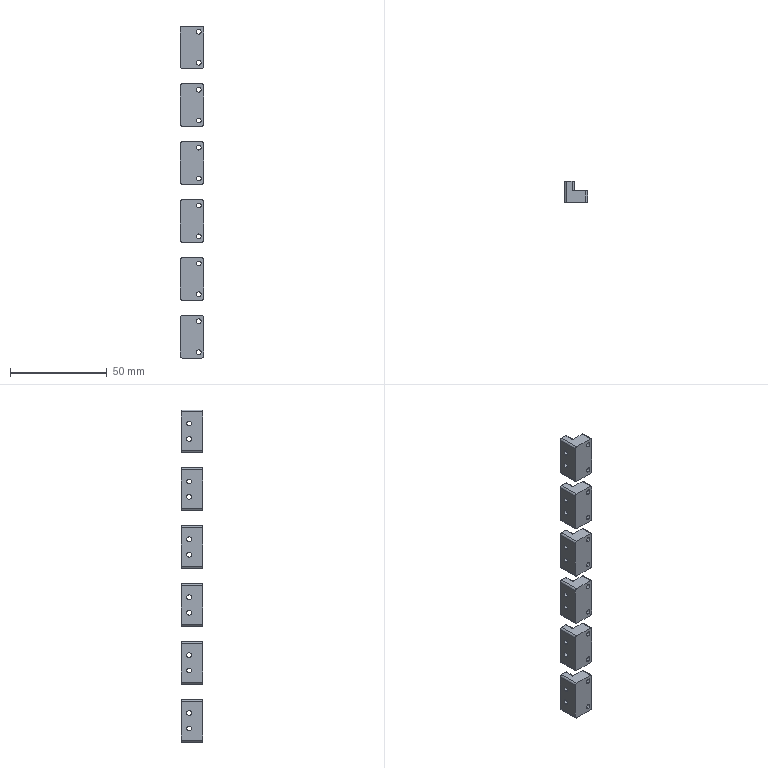CAM job | Mastercam | mm | 12 operations | part box 12 x 11 x 172
1. Facing | 20 - 63 平铣刀
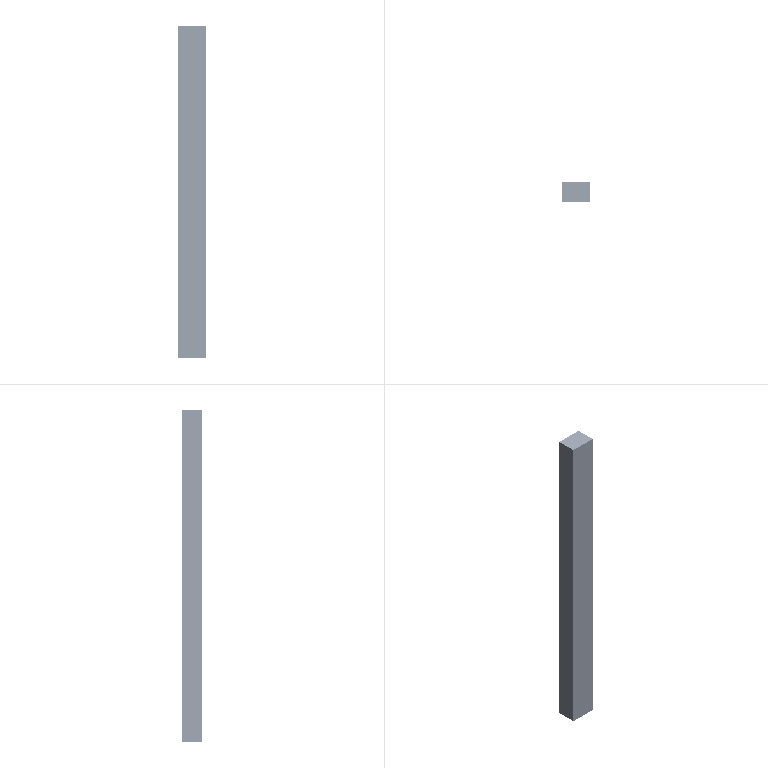2. Contour (Ramp) | 6 - 6 平铣刀
3. Contour (2D) | 6 - 6 平铣刀
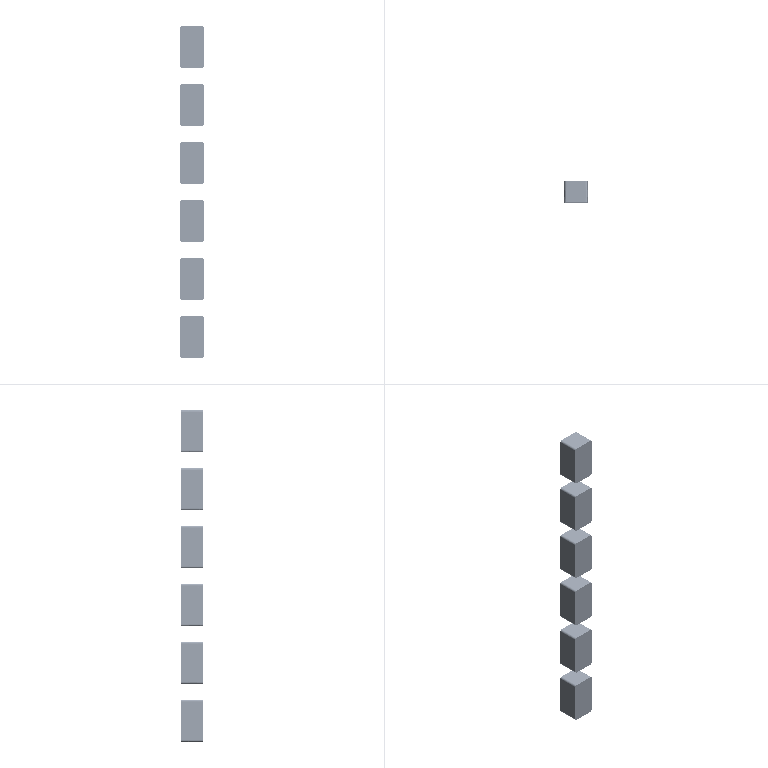4. Contour (2D chamfer) | 7 - 4 倒角刀
5. Drill/Counterbore | 7 - 4 倒角刀
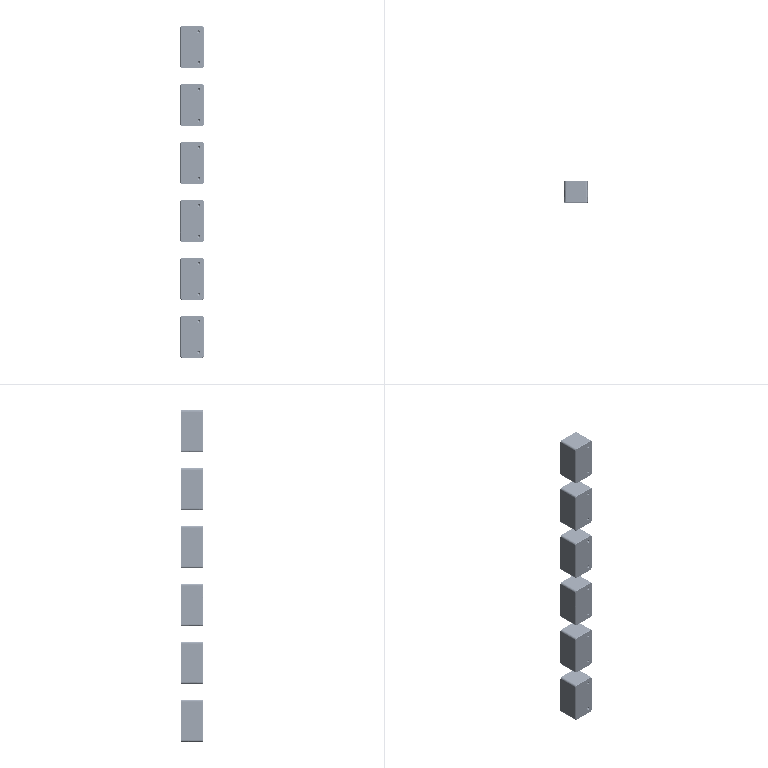6. Facing | 10 - 10 平铣刀
7. Drill/Counterbore | 7 - 4 倒角刀
8. Facing | 12 - 12 平铣刀
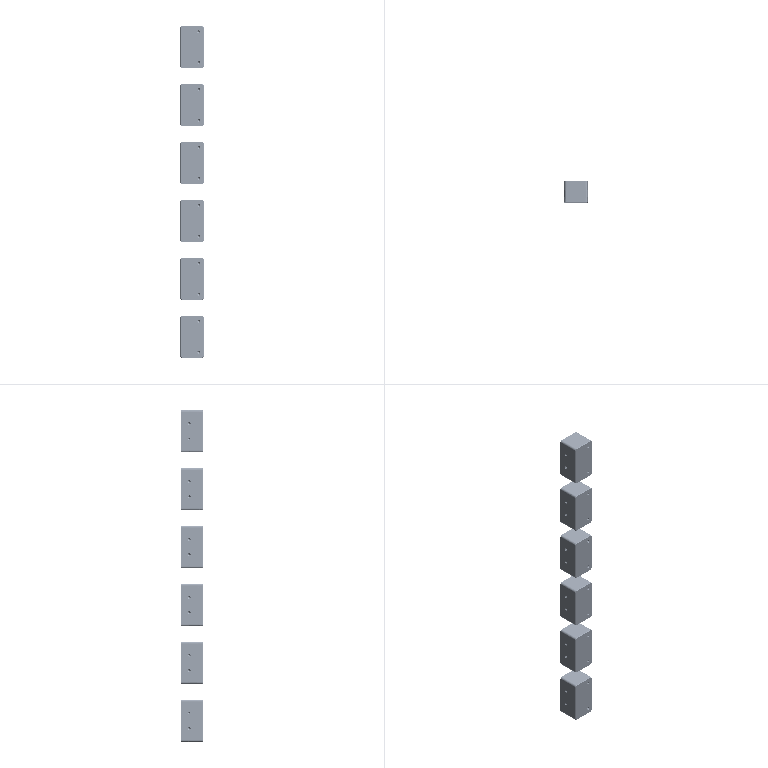9. Contour (Ramp) | 8 - 8 平铣刀
10. Contour (2D) | 8 - 8 平铣刀
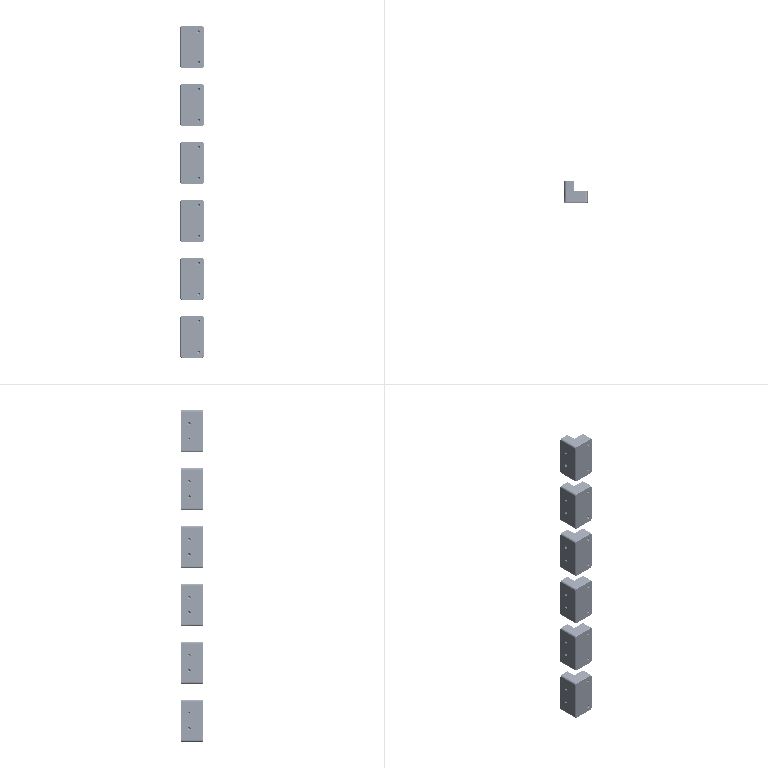11. Contour (2D) | 6 - 6 平铣刀
12. Model Chamfer | 7 - 4 倒角刀